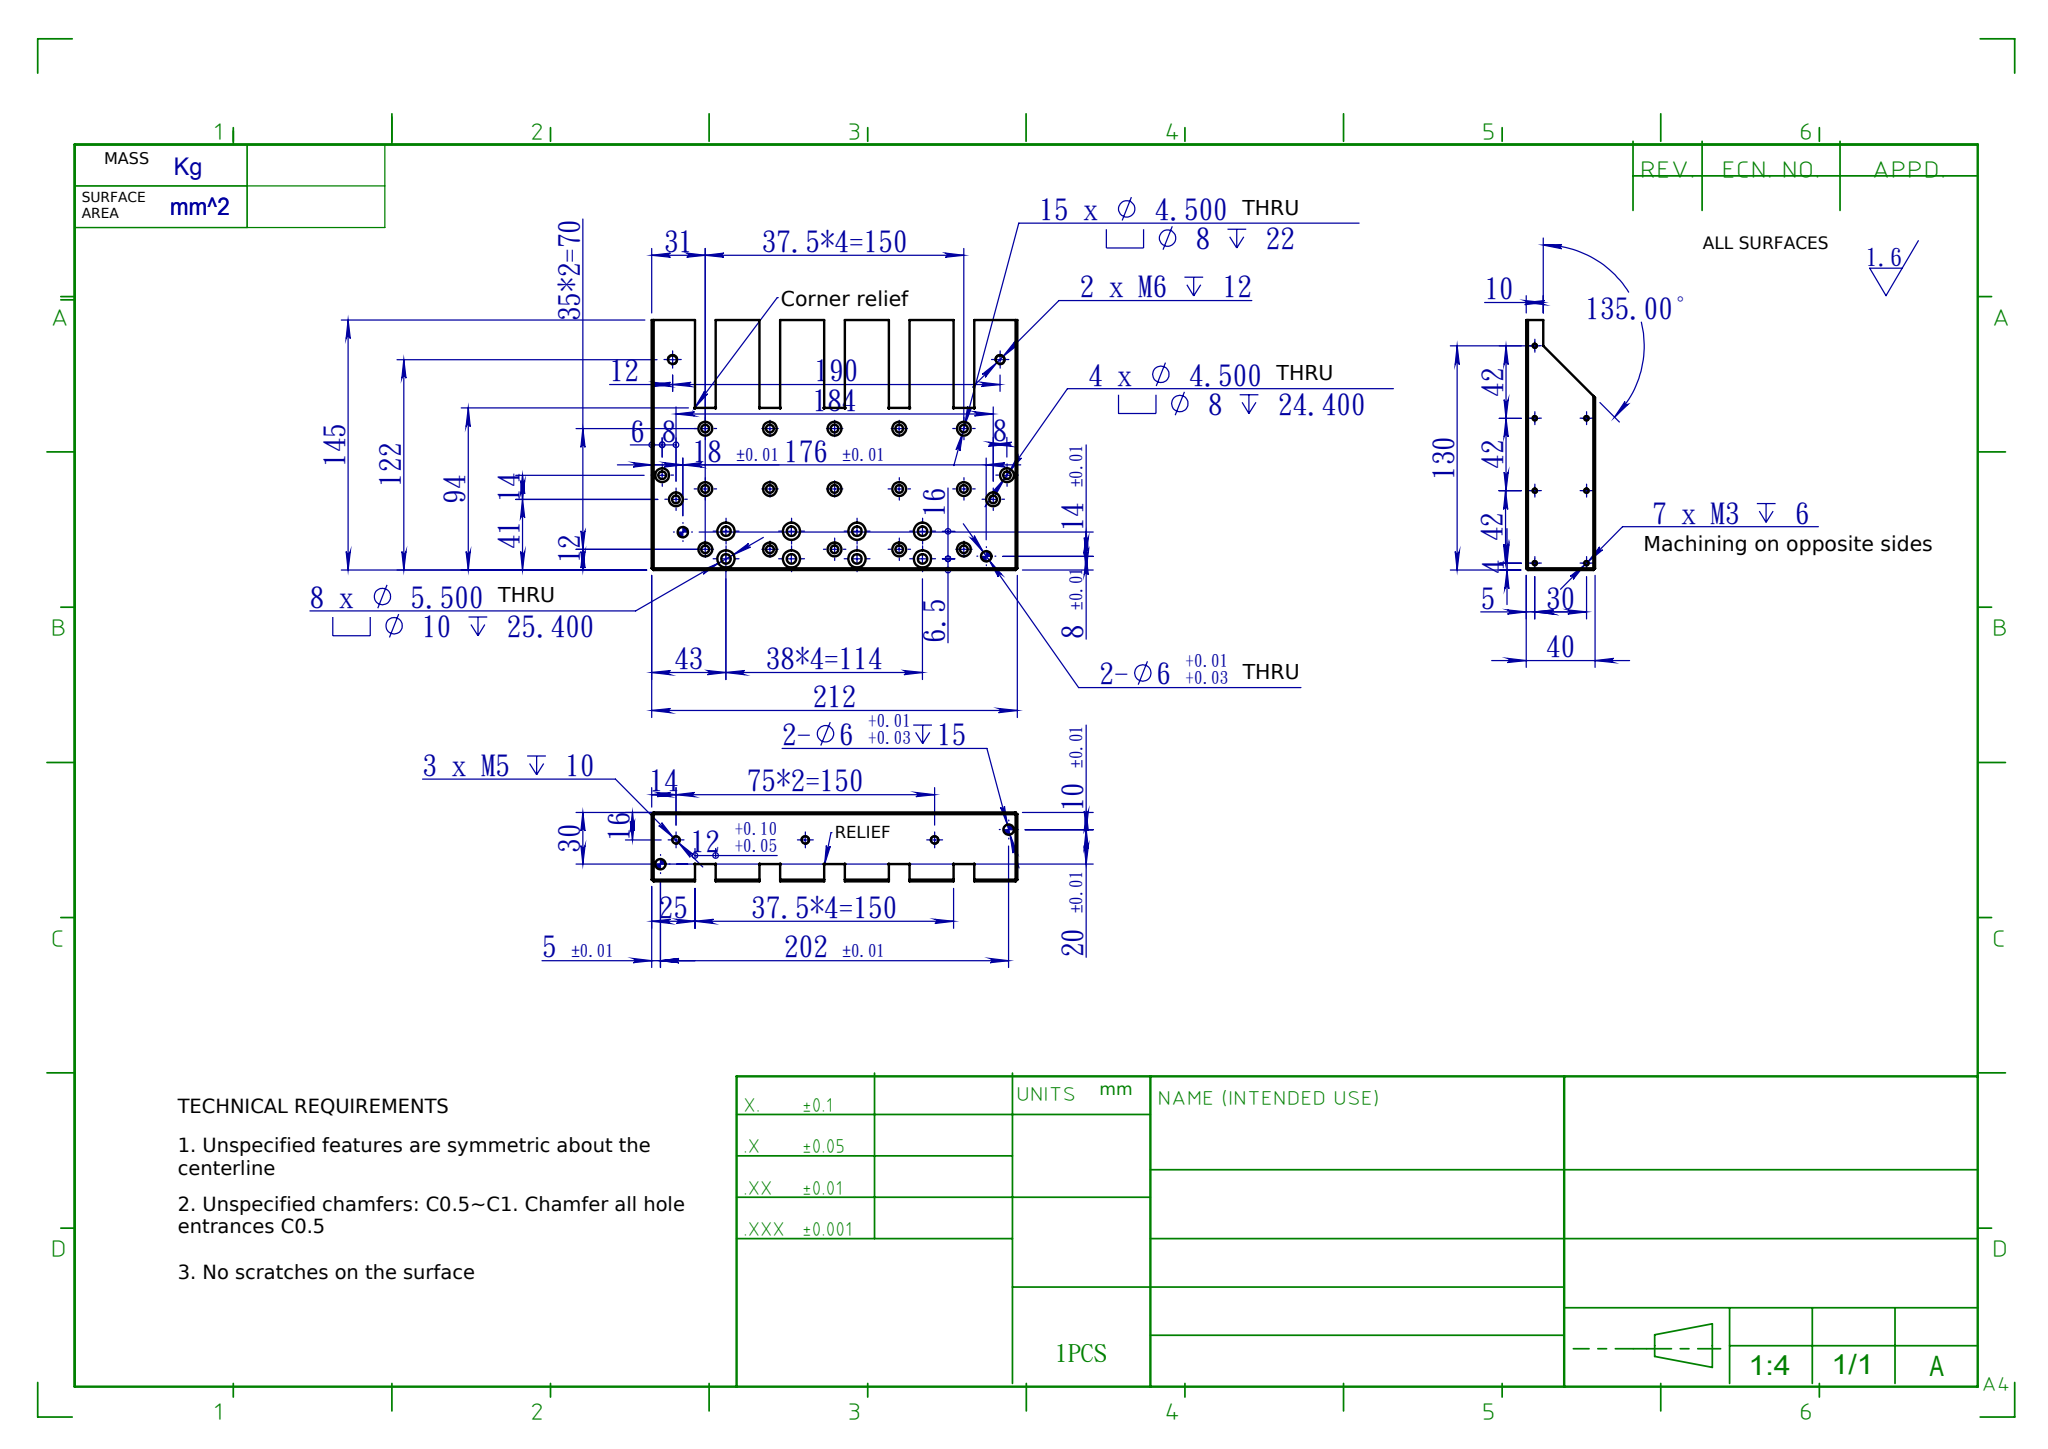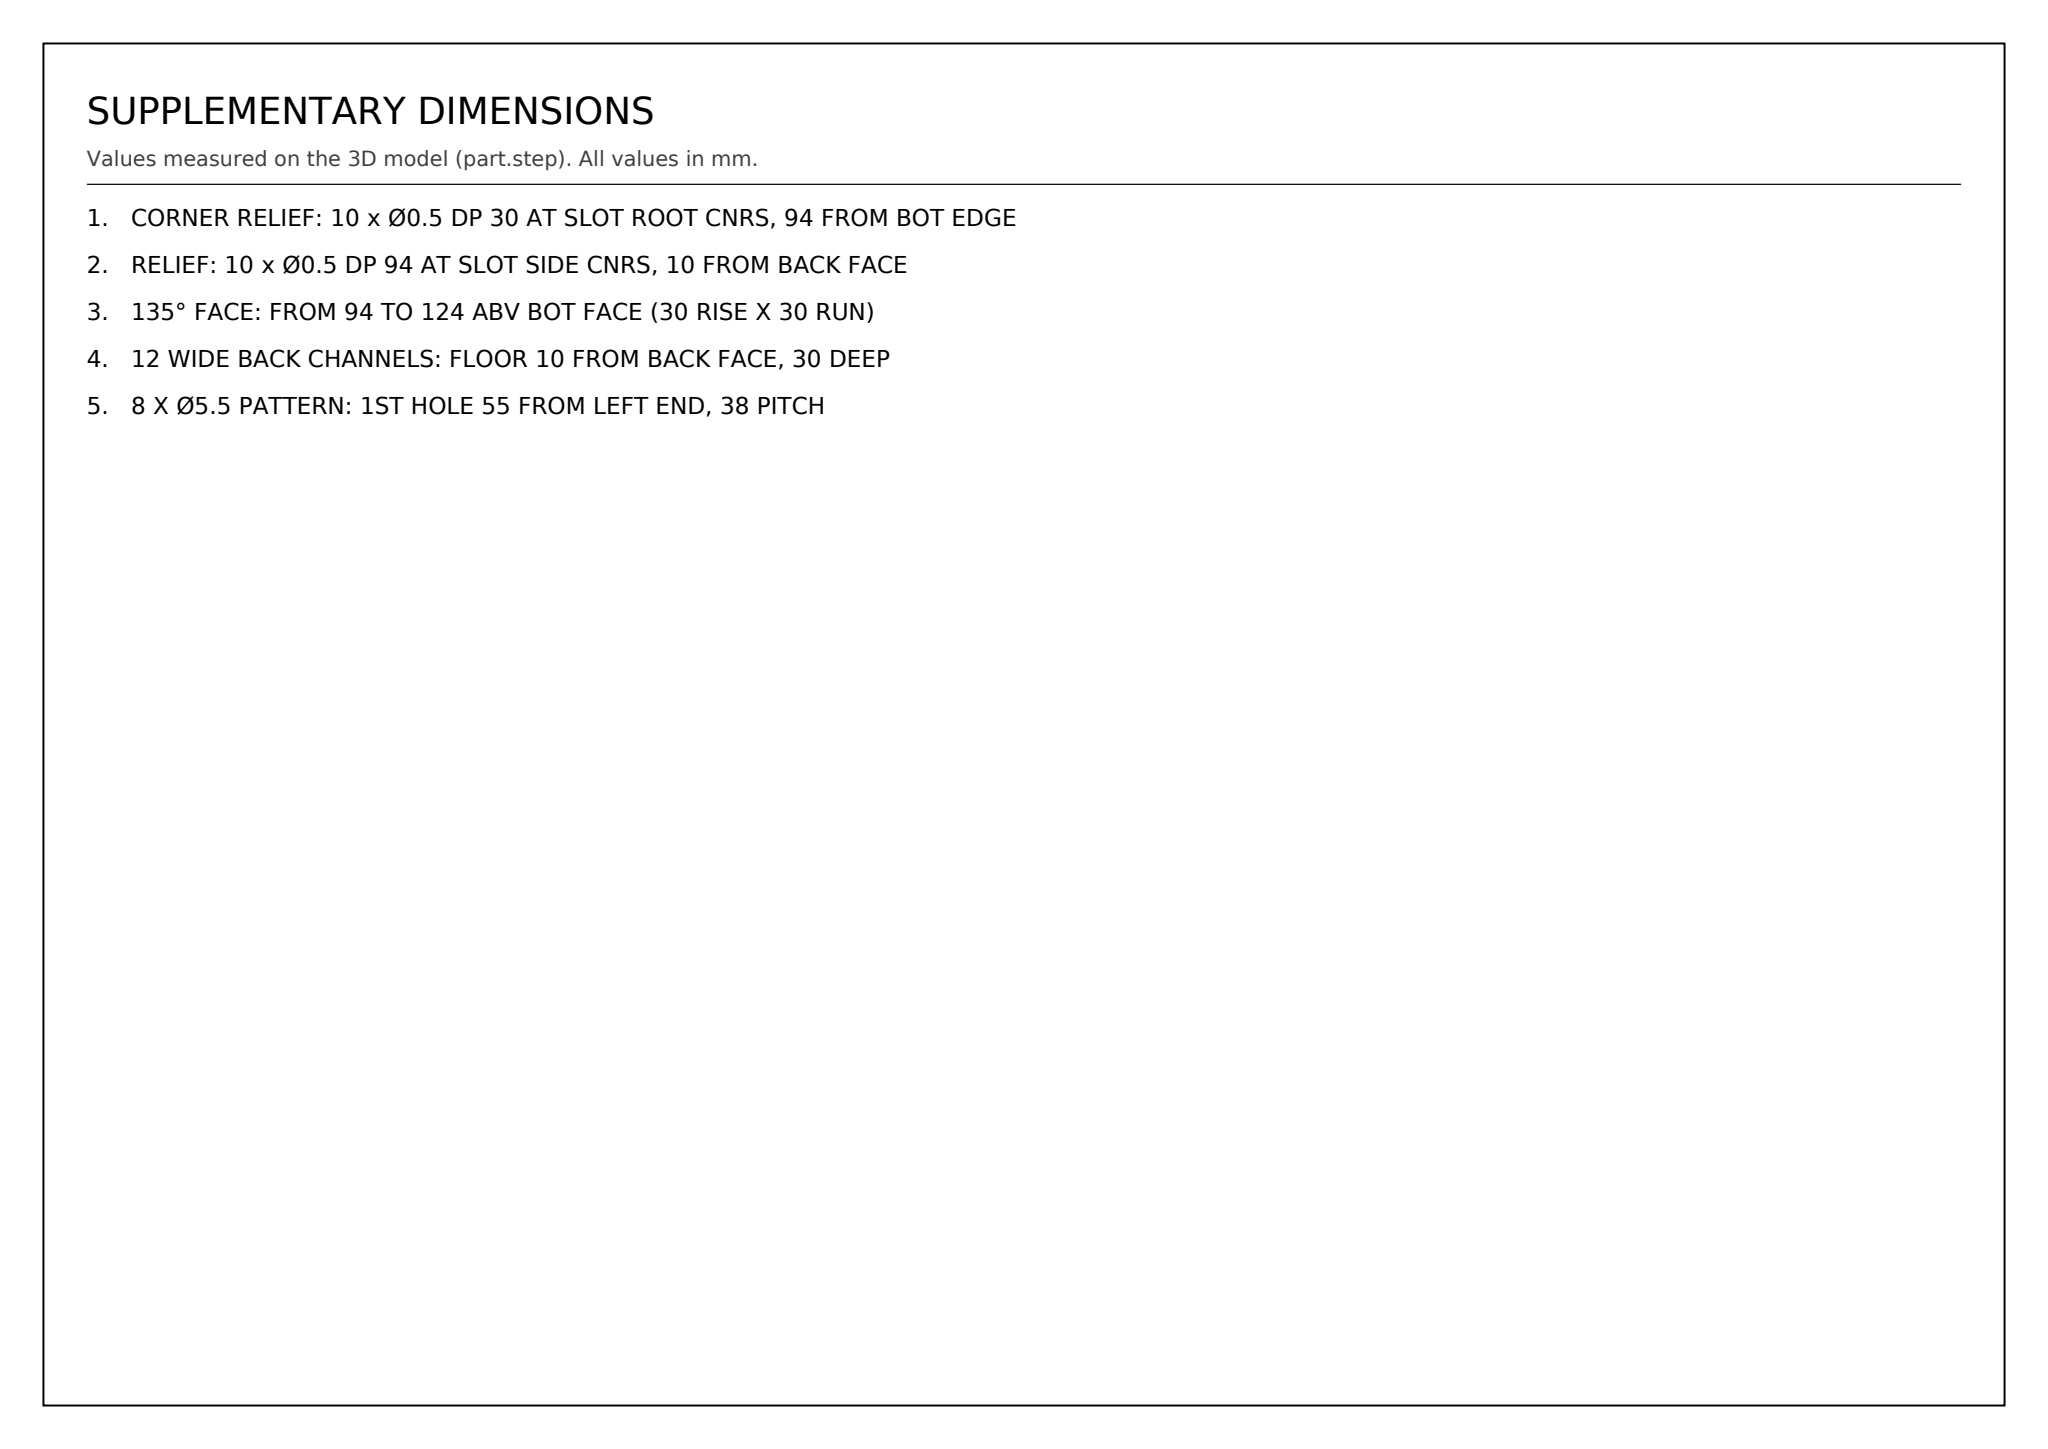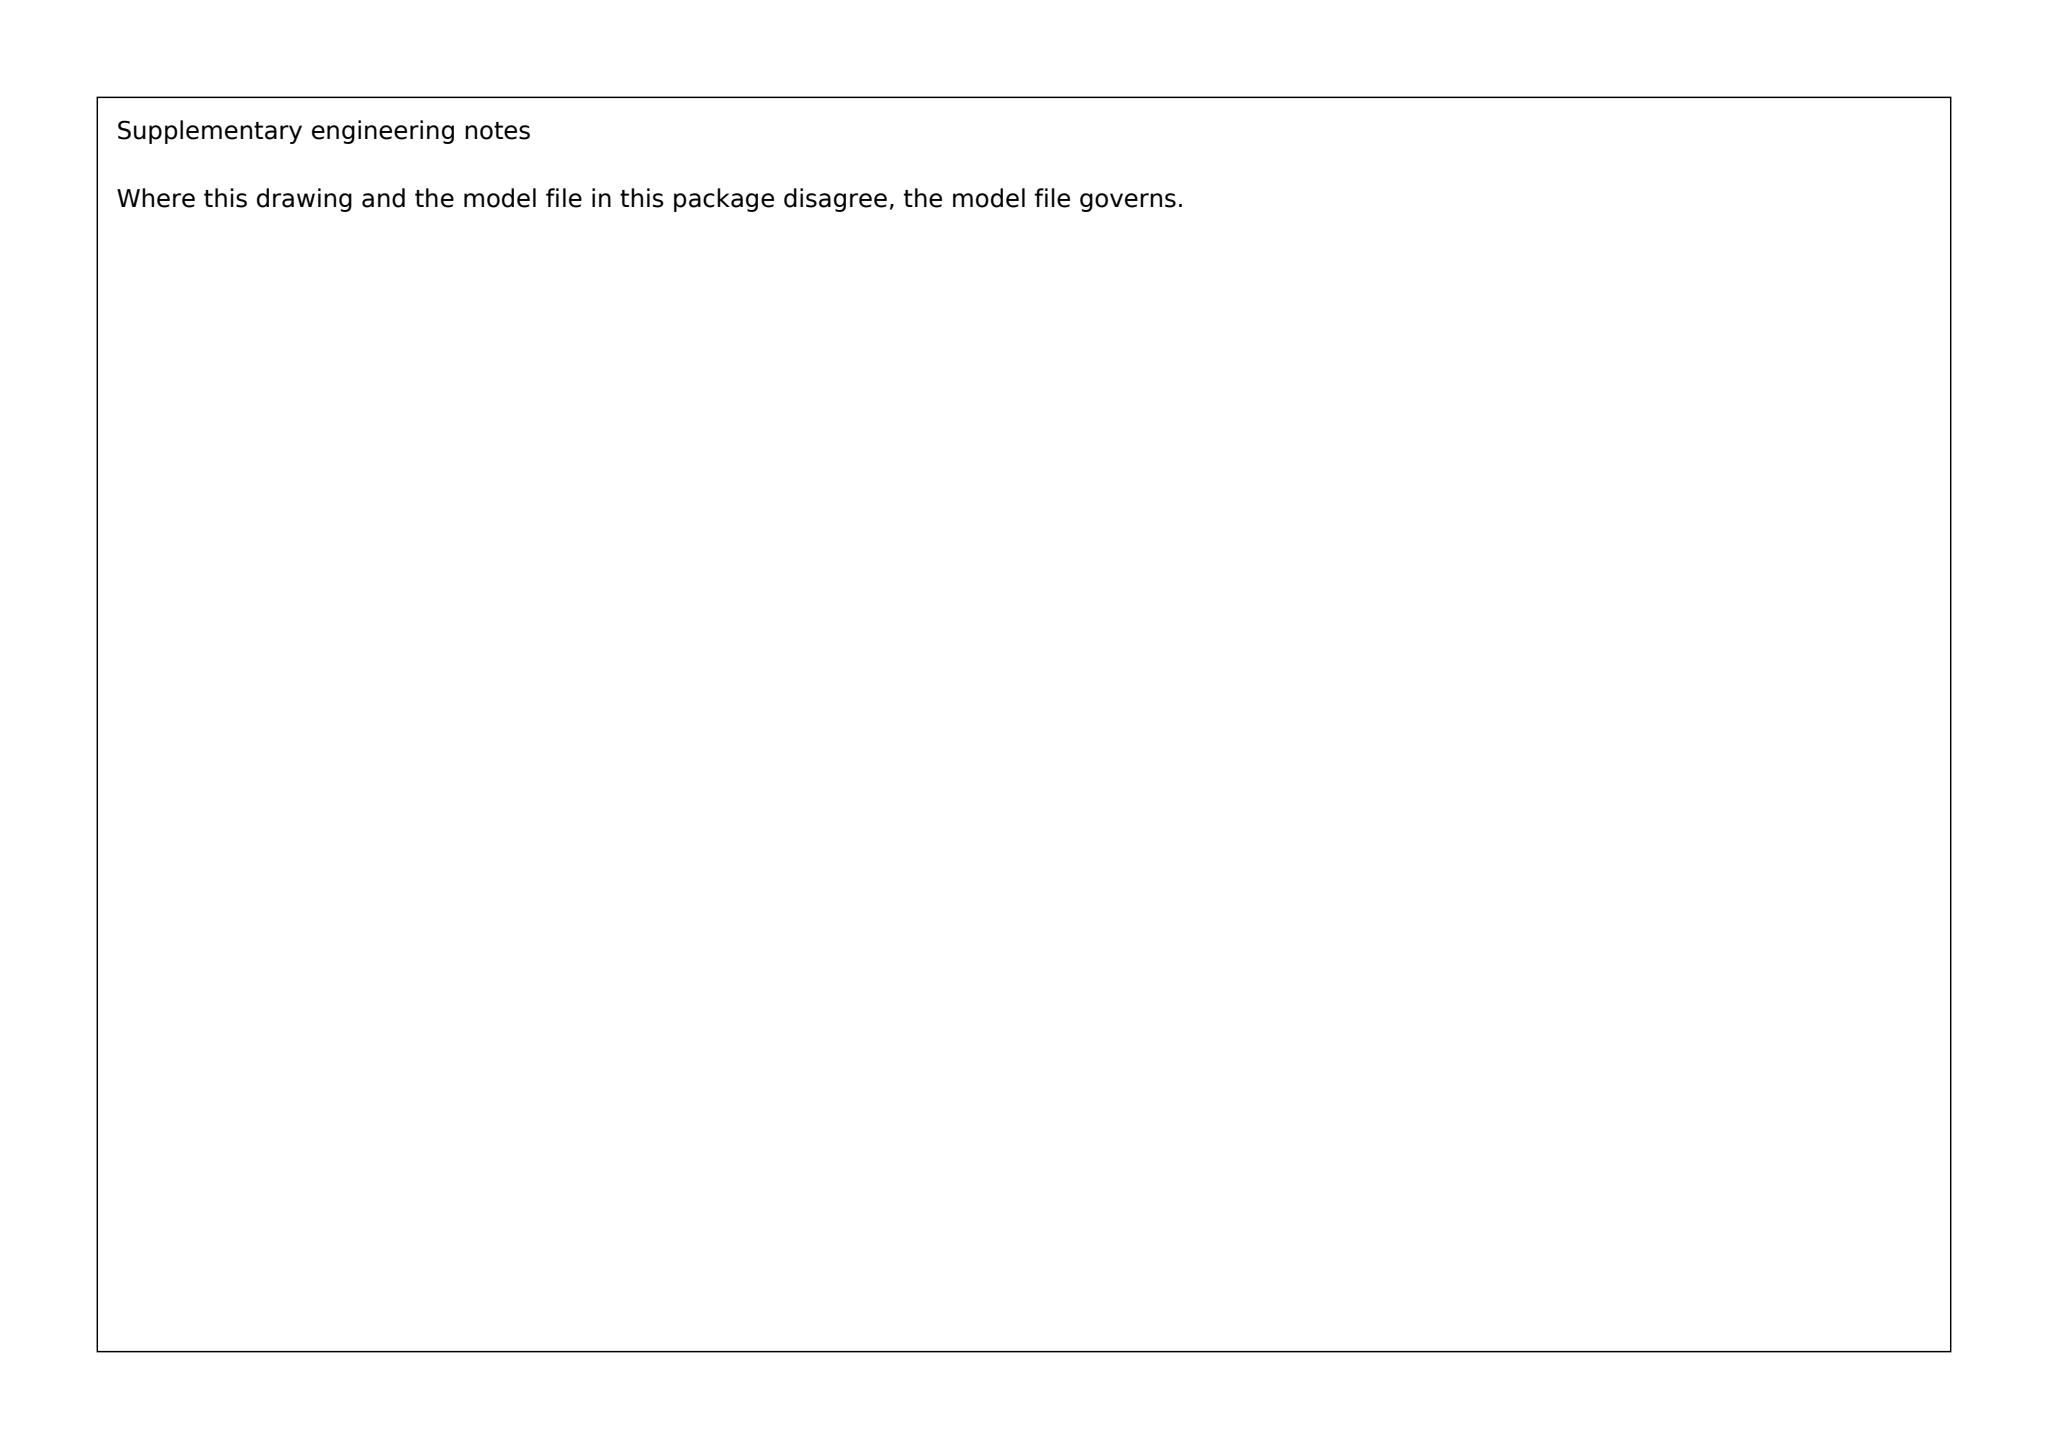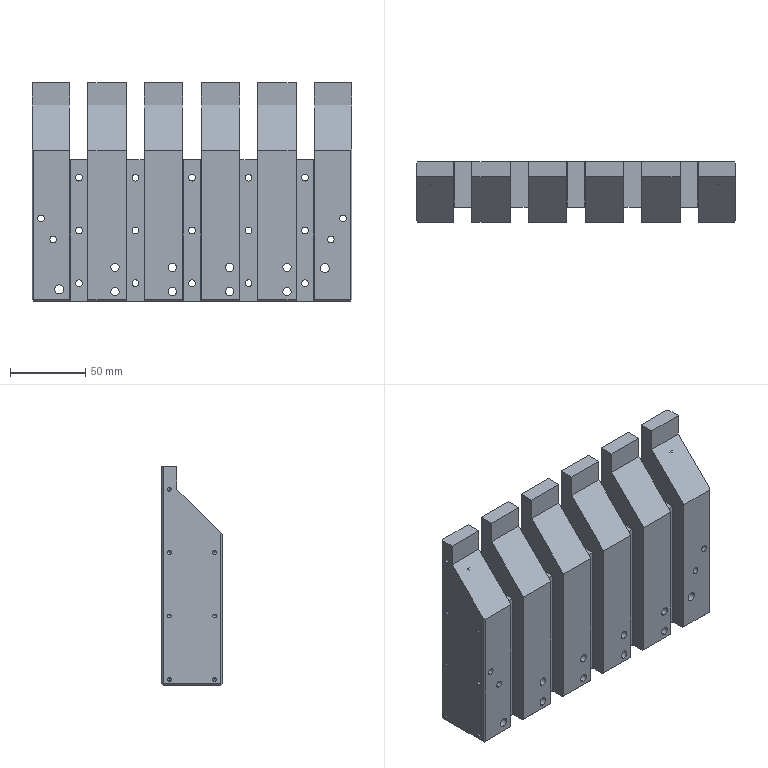Part | SolidWorks | mm | 1 solid | 336 faces | box 212 x 40 x 145 mm | volume 865440 mm3 | cylinder 184 | plane 114 | cone 38 | commonest cylinder face diameters 8 x38 4.5 x38 0.5 x30 2.5 x28 10 x16 5.5 x16 6 x8 4.2 x6
Drawing notes:
CORNER RELIEF: 10 x Ø0.5 DP 30 AT SLOT ROOT CNRS, 94 FROM BOT EDGE | from the solid: cyl Ø0.5 axis Y, len 30 (y10-40), z=94, x=25,37,62.5,74.5,100,112,137.5,149.5,175,187
RELIEF: 10 x Ø0.5 DP 94 AT SLOT SIDE CNRS, 10 FROM BACK FACE | from the solid: cyl Ø0.5 axis Z, len 94 (z0-94), y=10, same 10 x positions 25...187
135° FACE: FROM 94 TO 124 ABV BOT FACE (30 RISE X 30 RUN) | from the solid: y planes 10 & 40 (thk 10 upper / 40 lower), z plane 94 at base top; 135° slope gives end at z=94+30=124, bbox Z=145
12 WIDE BACK CHANNELS: FLOOR 10 FROM BACK FACE, 30 DEEP | from the solid: axis plane y=10 (15 faces) with edges at x=25/37, 62.5/74.5, 100/112, 137.5/149.5, 175/187 running z=0 to 94; part thk 40
8 X Ø5.5 PATTERN: 1ST HOLE 55 FROM LEFT END, 38 PITCH | from the solid: Ø5.5 cyls at x=55, 93, 131, 169 (z=6.5 & 22.5), bbox X=212
build123d program:
from build123d import *

# Parameters (mm, degrees)
SKETCH1_2_W                                          = 212
SKETCH1_2_H                                          = 40
BOSS_EXTRUDE1_DEPTH                                  = 145
SKETCH2_2_W                                          = 212
SKETCH2_2_H                                          = 15
CUT_EXTRUDE1_2_DEPTH                                 = 30
CUT_EXTRUDE3_DEPTH                                   = 258.622
SKETCH6_2_W                                          = 12
SKETCH6_2_H                                          = 100
CUT_EXTRUDE4_DEPTH                                   = 185.014
LINEAR_PATTERN1_COUNT                                = 5
LINEAR_PATTERN1_PITCH                                = 37.5
SKETCH9_2_R                                          = 3
CUT_EXTRUDE7_DEPTH                                   = 15
COUNTERBORE_FOR_M5_HEX_SOCKET_HEAD_CAP_S_D           = 5.5
COUNTERBORE_FOR_M5_HEX_SOCKET_HEAD_CAP_S_CBORE_D     = 10
COUNTERBORE_FOR_M5_HEX_SOCKET_HEAD_CAP_S_CBORE_DEPTH = 25.4
SKETCH3_R                                            = 3
CUT_EXTRUDE1_DEPTH                                   = 185.014
M5_TAPPED_HOLE1_D                                    = 4.2
M5_TAPPED_HOLE1_DEPTH                                = 12.4
M5_TAPPED_HOLE1_TIP                                  = 1.262
M3_TAPPED_HOLE1_AT_2_COUNT                           = 2
M3_TAPPED_HOLE1_AT_2_PITCH                           = 42
M3_TAPPED_HOLE1_AT_3_COUNT                           = 2
M3_TAPPED_HOLE1_AT_3_PITCH                           = 84
M3_TAPPED_HOLE1_AT_4_COUNT                           = 2
M3_TAPPED_HOLE1_AT_4_PITCH                           = 126
M3_TAPPED_HOLE1_AT_5_COUNT                           = 2
M3_TAPPED_HOLE1_AT_5_PITCH                           = 129.522
M3_TAPPED_HOLE1_AT_6_COUNT                           = 2
M3_TAPPED_HOLE1_AT_6_PITCH                           = 89.196
M3_TAPPED_HOLE1_AT_7_COUNT                           = 2
M3_TAPPED_HOLE1_AT_7_PITCH                           = 51.614
CBORE_FOR_M4_HEX_SOCKET_HEAD_CAP_SCREW1_D            = 4.5
CBORE_FOR_M4_HEX_SOCKET_HEAD_CAP_SCREW1_CBORE_D      = 8
CBORE_FOR_M4_HEX_SOCKET_HEAD_CAP_SCREW1_CBORE_DEPTH  = 24.4
M6_TAPPED_HOLE1_D                                    = 5
M6_TAPPED_HOLE1_DEPTH                                = 15
M6_TAPPED_HOLE1_TIP                                  = 1.502
CHAMFER1_SIZE                                        = 1
SKETCH10_2_W                                         = 12
SKETCH10_2_H                                         = 10
CUT_EXTRUDE8_DEPTH                                   = 144.08
SKETCH11_2_R                                         = 0.25
CUT_EXTRUDE9_DEPTH                                   = 94
COUNTERBORE_FOR_M4_HEX_SOCKET_HEAD_CAP_S_D           = 4.5
COUNTERBORE_FOR_M4_HEX_SOCKET_HEAD_CAP_S_CBORE_D     = 8
COUNTERBORE_FOR_M4_HEX_SOCKET_HEAD_CAP_S_CBORE_DEPTH = 22
CUT_EXTRUDE2_REACH                                   = 186.014
SKETCH12_R                                           = 0.25


with BuildPart() as part:
    # Sketch1_2 → Boss-Extrude1 (new body)
    with BuildSketch(Plane.XY):
        Rectangle(SKETCH1_2_W, SKETCH1_2_H)
    extrude(amount=BOSS_EXTRUDE1_DEPTH)

    # Sketch2_2 → Cut-Extrude1_2 (cut)
    with BuildSketch(Plane.XZ.offset(20)):
        with Locations((0, 137.5)):
            Rectangle(SKETCH2_2_W, SKETCH2_2_H)
    extrude(amount=-CUT_EXTRUDE1_2_DEPTH, mode=Mode.SUBTRACT)

    # Sketch4_2 → Cut-Extrude3 (cut, through all)
    with BuildSketch(Plane(origin=(106, 0, 0), x_dir=(0, 0, -1), z_dir=(1, 0, 0))):
        Polygon((-130, 10), (-100, -20), (-130, -20), align=None)
    extrude(amount=-CUT_EXTRUDE3_DEPTH, mode=Mode.SUBTRACT)

    # Sketch6_2 → Cut-Extrude4 (cut, through all)
    with BuildSketch(Plane.XZ.offset(20)):
        with Locations((-75, 144)):
            Rectangle(SKETCH6_2_W, SKETCH6_2_H)
    cut_extrude4 = extrude(amount=-CUT_EXTRUDE4_DEPTH, mode=Mode.SUBTRACT)

    # Linear Pattern1: Cut-Extrude4 ×5
    with Locations(*[(i * LINEAR_PATTERN1_PITCH, 0, 0) for i in range(1, LINEAR_PATTERN1_COUNT)]):
        add(cut_extrude4, mode=Mode.SUBTRACT)

    # Sketch9_2 → Cut-Extrude7 (cut)
    with BuildSketch(Plane(origin=(0, 0, 0), x_dir=(-1, 0, 0), z_dir=(0, 0, -1))):
        with Locations((-101, -10)):
            Circle(SKETCH9_2_R)
        with Locations((101, 10)):
            Circle(SKETCH9_2_R)
    extrude(amount=-CUT_EXTRUDE7_DEPTH, mode=Mode.SUBTRACT)

    # Counterbore for M5 Hex Socket Head Cap S (through all)
    with Locations(Plane(origin=(0, 20, 0), x_dir=(1, 0, 0), z_dir=(0, 1, 0))):
        with Locations((-51, -6.5), (-51, -22.5), (-13, -6.5), (-13, -22.5), (25, -22.5), (25, -6.5), (63, -6.5), (63, -22.5)):
            CounterBoreHole(COUNTERBORE_FOR_M5_HEX_SOCKET_HEAD_CAP_S_D / 2, COUNTERBORE_FOR_M5_HEX_SOCKET_HEAD_CAP_S_CBORE_D / 2, COUNTERBORE_FOR_M5_HEX_SOCKET_HEAD_CAP_S_CBORE_DEPTH)

    # Sketch3 → Cut-Extrude1 (cut, through all)
    with BuildSketch(Plane(origin=(0, 20, 0), x_dir=(1, 0, 0), z_dir=(0, 1, 0))):
        with Locations(Location((-88, -8, 0), (0, 0, 180))):
            Circle(SKETCH3_R)
        with Locations(Location((88, -22, 0), (0, 0, 180))):
            Circle(SKETCH3_R)
    extrude(amount=-CUT_EXTRUDE1_DEPTH, mode=Mode.SUBTRACT)

    # M5 Tapped Hole1
    with Locations(Plane(origin=(0, 0, 0), x_dir=(-1, 0, 0), z_dir=(0, 0, -1))):
        with Locations((-92, 4), (-17, 4), (58, 4)):
            Hole(M5_TAPPED_HOLE1_D / 2, depth=M5_TAPPED_HOLE1_DEPTH)
            with Locations((0, 0, -(M5_TAPPED_HOLE1_DEPTH + M5_TAPPED_HOLE1_TIP / 2))):  # 118° drill point
                Cone(0, M5_TAPPED_HOLE1_D / 2, M5_TAPPED_HOLE1_TIP, mode=Mode.SUBTRACT)

    # Sketch6 → M3 Tapped Hole1 (revolve, cut)
    with BuildSketch(Plane(origin=(106, 15, 130), x_dir=(0, 0, -1), z_dir=(0, 1, 0))):
        Polygon((0, 0), (0, 8.251), (1.25, 7.5), (1.25, 0), align=None)
    m3_tapped_hole1 = revolve(axis=Axis((112.35, 15, 130), (-1, 0, 0)), mode=Mode.SUBTRACT)

    # M3 Tapped Hole1 at 2: M3 Tapped Hole1 ×2
    with Locations(*[(0, 0, -i * M3_TAPPED_HOLE1_AT_2_PITCH) for i in range(1, M3_TAPPED_HOLE1_AT_2_COUNT)]):
        add(m3_tapped_hole1, mode=Mode.SUBTRACT)

    # M3 Tapped Hole1 at 3: M3 Tapped Hole1 ×2
    with Locations(*[(0, 0, -i * M3_TAPPED_HOLE1_AT_3_PITCH) for i in range(1, M3_TAPPED_HOLE1_AT_3_COUNT)]):
        add(m3_tapped_hole1, mode=Mode.SUBTRACT)

    # M3 Tapped Hole1 at 4: M3 Tapped Hole1 ×2
    with Locations(*[(0, 0, -i * M3_TAPPED_HOLE1_AT_4_PITCH) for i in range(1, M3_TAPPED_HOLE1_AT_4_COUNT)]):
        add(m3_tapped_hole1, mode=Mode.SUBTRACT)

    # M3 Tapped Hole1 at 5: M3 Tapped Hole1 ×2
    with Locations(*[Vector(0, -0.2316, -0.9728) * (i * M3_TAPPED_HOLE1_AT_5_PITCH) for i in range(1, M3_TAPPED_HOLE1_AT_5_COUNT)]):
        add(m3_tapped_hole1, mode=Mode.SUBTRACT)

    # M3 Tapped Hole1 at 6: M3 Tapped Hole1 ×2
    with Locations(*[Vector(0, -0.3363, -0.9417) * (i * M3_TAPPED_HOLE1_AT_6_PITCH) for i in range(1, M3_TAPPED_HOLE1_AT_6_COUNT)]):
        add(m3_tapped_hole1, mode=Mode.SUBTRACT)

    # M3 Tapped Hole1 at 7: M3 Tapped Hole1 ×2
    with Locations(*[Vector(0, -0.5812, -0.8137) * (i * M3_TAPPED_HOLE1_AT_7_PITCH) for i in range(1, M3_TAPPED_HOLE1_AT_7_COUNT)]):
        add(m3_tapped_hole1, mode=Mode.SUBTRACT)

    # Mirror1: M3 Tapped Hole1 across plane
    add(m3_tapped_hole1.mirror(Plane(origin=(0, 0, 0), x_dir=(0, 0, 1), z_dir=(1, 0, 0))), mode=Mode.SUBTRACT)

    # Mirror1 copy 1 sketch → Mirror1 copy 1 (revolve, cut)
    with BuildSketch(Plane(origin=(-106, 15, 88), x_dir=(0, 0, -1), z_dir=(0, 1, 0))):
        Polygon((0, 0), (0, -8.251), (1.25, -7.5), (1.25, 0), align=None)
    revolve(axis=Axis((-112.35, 15, 88), (-1, 0, 0)), mode=Mode.SUBTRACT)

    # Mirror1 copy 2 sketch → Mirror1 copy 2 (revolve, cut)
    with BuildSketch(Plane(origin=(-106, 15, 46), x_dir=(0, 0, -1), z_dir=(0, 1, 0))):
        Polygon((0, 0), (0, -8.251), (1.25, -7.5), (1.25, 0), align=None)
    revolve(axis=Axis((-112.35, 15, 46), (-1, 0, 0)), mode=Mode.SUBTRACT)

    # Mirror1 copy 3 sketch → Mirror1 copy 3 (revolve, cut)
    with BuildSketch(Plane(origin=(-106, 15, 4), x_dir=(0, 0, -1), z_dir=(0, 1, 0))):
        Polygon((0, 0), (0, -8.251), (1.25, -7.5), (1.25, 0), align=None)
    revolve(axis=Axis((-112.35, 15, 4), (-1, 0, 0)), mode=Mode.SUBTRACT)

    # Mirror1 copy 4 sketch → Mirror1 copy 4 (revolve, cut)
    with BuildSketch(Plane(origin=(-106, -15, 4), x_dir=(0, 0, -1), z_dir=(0, 1, 0))):
        Polygon((0, 0), (0, -8.251), (1.25, -7.5), (1.25, 0), align=None)
    revolve(axis=Axis((-112.35, -15, 4), (-1, 0, 0)), mode=Mode.SUBTRACT)

    # Mirror1 copy 5 sketch → Mirror1 copy 5 (revolve, cut)
    with BuildSketch(Plane(origin=(-106, -15, 46), x_dir=(0, 0, -1), z_dir=(0, 1, 0))):
        Polygon((0, 0), (0, -8.251), (1.25, -7.5), (1.25, 0), align=None)
    revolve(axis=Axis((-112.35, -15, 46), (-1, 0, 0)), mode=Mode.SUBTRACT)

    # Mirror1 copy 6 sketch → Mirror1 copy 6 (revolve, cut)
    with BuildSketch(Plane(origin=(-106, -15, 88), x_dir=(0, 0, -1), z_dir=(0, 1, 0))):
        Polygon((0, 0), (0, -8.251), (1.25, -7.5), (1.25, 0), align=None)
    revolve(axis=Axis((-112.35, -15, 88), (-1, 0, 0)), mode=Mode.SUBTRACT)

    # CBORE for M4 Hex Socket Head Cap Screw1 (through all)
    with Locations(Plane(origin=(0, 20, 0), x_dir=(1, 0, 0), z_dir=(0, 1, 0))):
        with Locations((-92, -41), (-100, -55), (100, -55), (92, -41)):
            CounterBoreHole(CBORE_FOR_M4_HEX_SOCKET_HEAD_CAP_SCREW1_D / 2, CBORE_FOR_M4_HEX_SOCKET_HEAD_CAP_SCREW1_CBORE_D / 2, CBORE_FOR_M4_HEX_SOCKET_HEAD_CAP_SCREW1_CBORE_DEPTH)

    # M6 Tapped Hole1
    with Locations(Plane(origin=(0, 20, 0), x_dir=(1, 0, 0), z_dir=(0, 1, 0))):
        with Locations((94, -122), (-96, -122)):
            Hole(M6_TAPPED_HOLE1_D / 2, depth=M6_TAPPED_HOLE1_DEPTH)
            with Locations((0, 0, -(M6_TAPPED_HOLE1_DEPTH + M6_TAPPED_HOLE1_TIP / 2))):  # 118° drill point
                Cone(0, M6_TAPPED_HOLE1_D / 2, M6_TAPPED_HOLE1_TIP, mode=Mode.SUBTRACT)

    # Chamfer1
    chamfer1_edges = [part.edges().sort_by_distance(p)[0] for p in [
        (106, -20, 50),
        (-106, -20, 50),
        (0, 20, 0),
        (106, 0, 0),
        (0, -20, 0),
        (-106, 0, 0),
        (-106, 20, 72.5),
        (106, 20, 72.5),
    ]]
    chamfer(chamfer1_edges, length=CHAMFER1_SIZE)

    # Sketch10_2 → Cut-Extrude8 (cut, through all)
    with BuildSketch(Plane.XY.offset(94)):
        with Locations((75, -15)):
            Rectangle(SKETCH10_2_W, SKETCH10_2_H)
        with Locations((37.5, -15)):
            Rectangle(SKETCH10_2_W, SKETCH10_2_H)
        with Locations((0, -15)):
            Rectangle(SKETCH10_2_W, SKETCH10_2_H)
        with Locations((-37.5, -15)):
            Rectangle(SKETCH10_2_W, SKETCH10_2_H)
        with Locations((-75, -15)):
            Rectangle(SKETCH10_2_W, SKETCH10_2_H)
    extrude(amount=-CUT_EXTRUDE8_DEPTH, mode=Mode.SUBTRACT)

    # Sketch11_2 → Cut-Extrude9 (cut)
    with BuildSketch(Plane(origin=(0, 0, 0), x_dir=(-1, 0, 0), z_dir=(0, 0, -1))):
        with Locations((-81, -10)):
            Circle(SKETCH11_2_R)
        with Locations((-69, -10)):
            Circle(SKETCH11_2_R)
        with Locations((-43.5, -10)):
            Circle(SKETCH11_2_R)
        with Locations((-31.5, -10)):
            Circle(SKETCH11_2_R)
        with Locations((-6, -10)):
            Circle(SKETCH11_2_R)
        with Locations((6, -10)):
            Circle(SKETCH11_2_R)
        with Locations((31.5, -10)):
            Circle(SKETCH11_2_R)
        with Locations((43.5, -10)):
            Circle(SKETCH11_2_R)
        with Locations((69, -10)):
            Circle(SKETCH11_2_R)
        with Locations((81, -10)):
            Circle(SKETCH11_2_R)
    extrude(amount=-CUT_EXTRUDE9_DEPTH, mode=Mode.SUBTRACT)

    # Counterbore for M4 Hex Socket Head Cap S (through all)
    with Locations(Plane(origin=(0, 20, 0), x_dir=(1, 0, 0), z_dir=(0, 1, 0))):
        with Locations((75, -82), (75, -47), (75, -12), (37.5, -82), (37.5, -47), (37.5, -12), (0, -82), (0, -47), (0, -12), (-37.5, -82), (-37.5, -47), (-37.5, -12), (-75, -82), (-75, -47), (-75, -12)):
            CounterBoreHole(COUNTERBORE_FOR_M4_HEX_SOCKET_HEAD_CAP_S_D / 2, COUNTERBORE_FOR_M4_HEX_SOCKET_HEAD_CAP_S_CBORE_D / 2, COUNTERBORE_FOR_M4_HEX_SOCKET_HEAD_CAP_S_CBORE_DEPTH)

    # Cut-Extrude2: up to this face of the body (flat: up to its plane)
    cut_extrude2_end = Plane(part.part.faces().sort_by_distance((37.5, -10, 93.053))[0])
    # Sketch12 → Cut-Extrude2 (cut, up to the picked face)
    with BuildSketch(Plane(origin=(0, 20, 0), x_dir=(1, 0, 0), z_dir=(0, 1, 0)), mode=Mode.PRIVATE) as cut_extrude2_sk1:
        with Locations((-81, -94)):
            Circle(SKETCH12_R)
    cut_extrude2_tool1 = split(extrude(cut_extrude2_sk1.sketch, amount=-CUT_EXTRUDE2_REACH, mode=Mode.PRIVATE), bisect_by=cut_extrude2_end, keep=Keep.BOTH, mode=Mode.PRIVATE)
    # Sketch12 → Cut-Extrude2 (cut, up to the picked face)
    with BuildSketch(Plane(origin=(0, 20, 0), x_dir=(1, 0, 0), z_dir=(0, 1, 0)), mode=Mode.PRIVATE) as cut_extrude2_sk2:
        with Locations((-69, -94)):
            Circle(SKETCH12_R)
    cut_extrude2_tool2 = split(extrude(cut_extrude2_sk2.sketch, amount=-CUT_EXTRUDE2_REACH, mode=Mode.PRIVATE), bisect_by=cut_extrude2_end, keep=Keep.BOTH, mode=Mode.PRIVATE)
    # Sketch12 → Cut-Extrude2 (cut, up to the picked face)
    with BuildSketch(Plane(origin=(0, 20, 0), x_dir=(1, 0, 0), z_dir=(0, 1, 0)), mode=Mode.PRIVATE) as cut_extrude2_sk3:
        with Locations((-43.5, -94)):
            Circle(SKETCH12_R)
    cut_extrude2_tool3 = split(extrude(cut_extrude2_sk3.sketch, amount=-CUT_EXTRUDE2_REACH, mode=Mode.PRIVATE), bisect_by=cut_extrude2_end, keep=Keep.BOTH, mode=Mode.PRIVATE)
    # Sketch12 → Cut-Extrude2 (cut, up to the picked face)
    with BuildSketch(Plane(origin=(0, 20, 0), x_dir=(1, 0, 0), z_dir=(0, 1, 0)), mode=Mode.PRIVATE) as cut_extrude2_sk4:
        with Locations((-31.5, -94)):
            Circle(SKETCH12_R)
    cut_extrude2_tool4 = split(extrude(cut_extrude2_sk4.sketch, amount=-CUT_EXTRUDE2_REACH, mode=Mode.PRIVATE), bisect_by=cut_extrude2_end, keep=Keep.BOTH, mode=Mode.PRIVATE)
    # Sketch12 → Cut-Extrude2 (cut, up to the picked face)
    with BuildSketch(Plane(origin=(0, 20, 0), x_dir=(1, 0, 0), z_dir=(0, 1, 0)), mode=Mode.PRIVATE) as cut_extrude2_sk5:
        with Locations((-6, -94)):
            Circle(SKETCH12_R)
    cut_extrude2_tool5 = split(extrude(cut_extrude2_sk5.sketch, amount=-CUT_EXTRUDE2_REACH, mode=Mode.PRIVATE), bisect_by=cut_extrude2_end, keep=Keep.BOTH, mode=Mode.PRIVATE)
    # Sketch12 → Cut-Extrude2 (cut, up to the picked face)
    with BuildSketch(Plane(origin=(0, 20, 0), x_dir=(1, 0, 0), z_dir=(0, 1, 0)), mode=Mode.PRIVATE) as cut_extrude2_sk6:
        with Locations((6, -94)):
            Circle(SKETCH12_R)
    cut_extrude2_tool6 = split(extrude(cut_extrude2_sk6.sketch, amount=-CUT_EXTRUDE2_REACH, mode=Mode.PRIVATE), bisect_by=cut_extrude2_end, keep=Keep.BOTH, mode=Mode.PRIVATE)
    # Sketch12 → Cut-Extrude2 (cut, up to the picked face)
    with BuildSketch(Plane(origin=(0, 20, 0), x_dir=(1, 0, 0), z_dir=(0, 1, 0)), mode=Mode.PRIVATE) as cut_extrude2_sk7:
        with Locations((31.5, -94)):
            Circle(SKETCH12_R)
    cut_extrude2_tool7 = split(extrude(cut_extrude2_sk7.sketch, amount=-CUT_EXTRUDE2_REACH, mode=Mode.PRIVATE), bisect_by=cut_extrude2_end, keep=Keep.BOTH, mode=Mode.PRIVATE)
    # Sketch12 → Cut-Extrude2 (cut, up to the picked face)
    with BuildSketch(Plane(origin=(0, 20, 0), x_dir=(1, 0, 0), z_dir=(0, 1, 0)), mode=Mode.PRIVATE) as cut_extrude2_sk8:
        with Locations((43.5, -94)):
            Circle(SKETCH12_R)
    cut_extrude2_tool8 = split(extrude(cut_extrude2_sk8.sketch, amount=-CUT_EXTRUDE2_REACH, mode=Mode.PRIVATE), bisect_by=cut_extrude2_end, keep=Keep.BOTH, mode=Mode.PRIVATE)
    # Sketch12 → Cut-Extrude2 (cut, up to the picked face)
    with BuildSketch(Plane(origin=(0, 20, 0), x_dir=(1, 0, 0), z_dir=(0, 1, 0)), mode=Mode.PRIVATE) as cut_extrude2_sk9:
        with Locations((69, -94)):
            Circle(SKETCH12_R)
    cut_extrude2_tool9 = split(extrude(cut_extrude2_sk9.sketch, amount=-CUT_EXTRUDE2_REACH, mode=Mode.PRIVATE), bisect_by=cut_extrude2_end, keep=Keep.BOTH, mode=Mode.PRIVATE)
    # Sketch12 → Cut-Extrude2 (cut, up to the picked face)
    with BuildSketch(Plane(origin=(0, 20, 0), x_dir=(1, 0, 0), z_dir=(0, 1, 0)), mode=Mode.PRIVATE) as cut_extrude2_sk10:
        with Locations((81, -94)):
            Circle(SKETCH12_R)
    cut_extrude2_tool10 = split(extrude(cut_extrude2_sk10.sketch, amount=-CUT_EXTRUDE2_REACH, mode=Mode.PRIVATE), bisect_by=cut_extrude2_end, keep=Keep.BOTH, mode=Mode.PRIVATE)
    add(cut_extrude2_tool1.solids().sort_by(Axis((-81, 20, 94), (0, -1, 0)))[0], mode=Mode.SUBTRACT)
    add(cut_extrude2_tool2.solids().sort_by(Axis((-69, 20, 94), (0, -1, 0)))[0], mode=Mode.SUBTRACT)
    add(cut_extrude2_tool3.solids().sort_by(Axis((-43.5, 20, 94), (0, -1, 0)))[0], mode=Mode.SUBTRACT)
    add(cut_extrude2_tool4.solids().sort_by(Axis((-31.5, 20, 94), (0, -1, 0)))[0], mode=Mode.SUBTRACT)
    add(cut_extrude2_tool5.solids().sort_by(Axis((-6, 20, 94), (0, -1, 0)))[0], mode=Mode.SUBTRACT)
    add(cut_extrude2_tool6.solids().sort_by(Axis((6, 20, 94), (0, -1, 0)))[0], mode=Mode.SUBTRACT)
    add(cut_extrude2_tool7.solids().sort_by(Axis((31.5, 20, 94), (0, -1, 0)))[0], mode=Mode.SUBTRACT)
    add(cut_extrude2_tool8.solids().sort_by(Axis((43.5, 20, 94), (0, -1, 0)))[0], mode=Mode.SUBTRACT)
    add(cut_extrude2_tool9.solids().sort_by(Axis((69, 20, 94), (0, -1, 0)))[0], mode=Mode.SUBTRACT)
    add(cut_extrude2_tool10.solids().sort_by(Axis((81, 20, 94), (0, -1, 0)))[0], mode=Mode.SUBTRACT)


solid = part.part